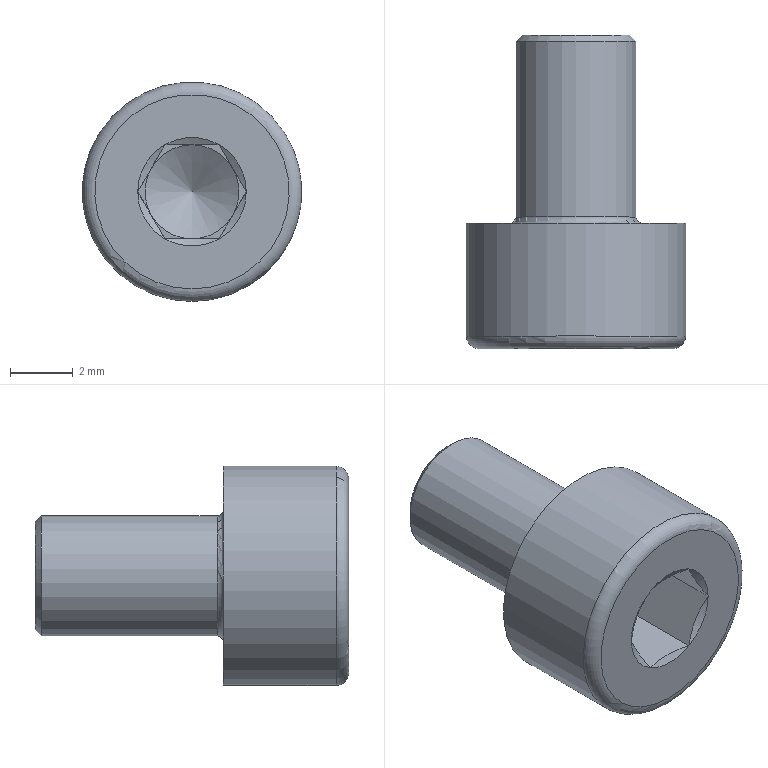Component | NX | SCREW_M4X6_2 | 1 solid | 27 faces | volume 200 mm3 | plane 15 | cone 8 | cylinder 2 | torus 2 | commonest cylinder face diameters 3.838 x1 7 x1